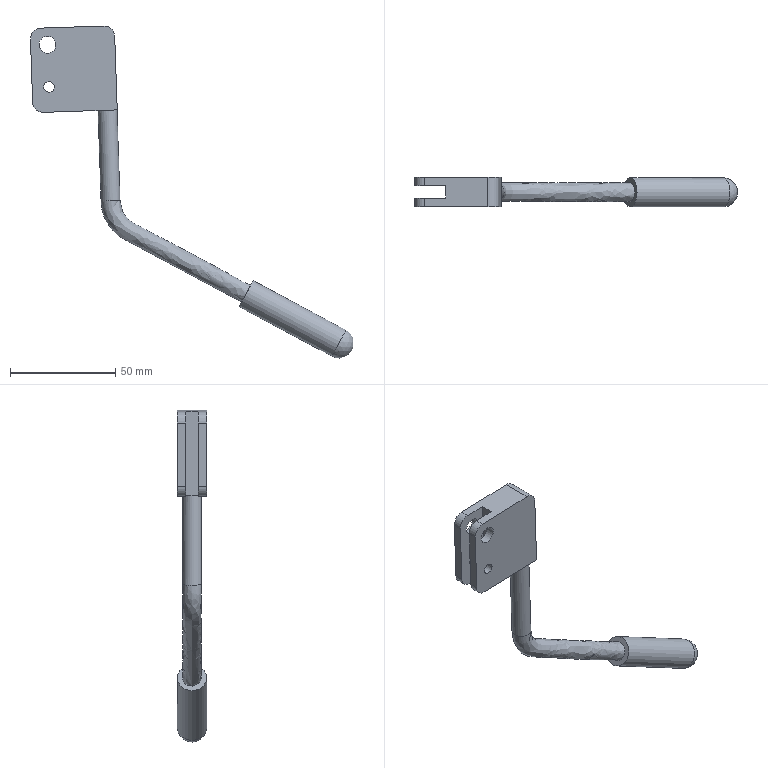Component | NX | HANDLE | 1 solid | 26 faces | volume 34363 mm3 | plane 13 | cylinder 11 | spline 1 | sphere 1 | commonest cylinder face diameters 10 x5 5 x2 8 x2 9 x1 14 x1